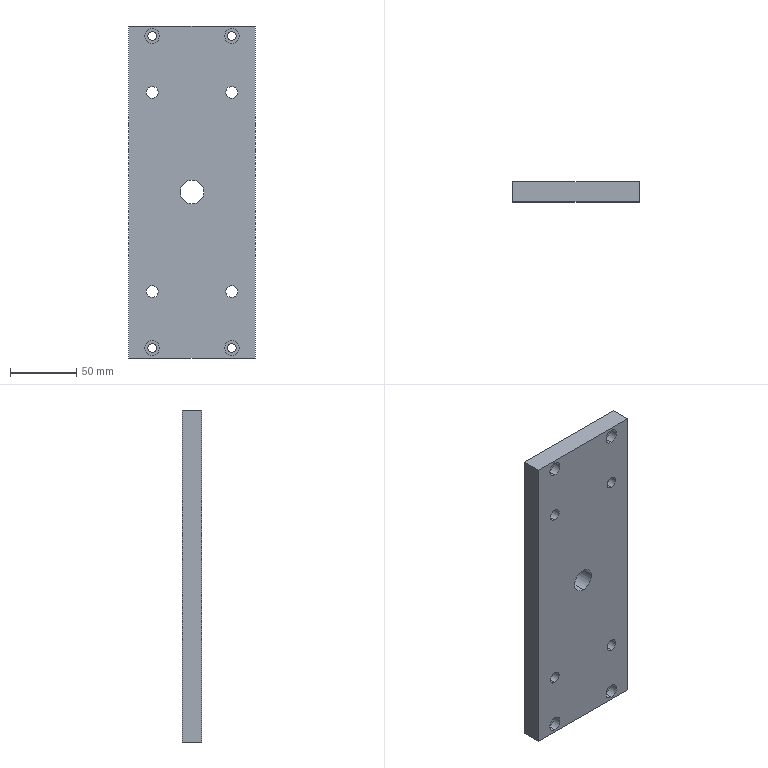Component | SolidWorks | 8TC-A15004-D0-01A-1 | 1 solid | 48 faces | box 95 x 15 x 250 mm | volume 341116 mm3 | cylinder 34 | plane 14 | commonest cylinder face diameters 15 x8 9 x8 11 x8 6.6 x8 18 x2 | material #45
build123d program:
from build123d import *

# Parameters (mm, degrees)
SKETCH1_W                                       = 95
SKETCH1_H                                       = 250
BOSS_EXTRUDE1_DEPTH                             = 7.5
M6_HEX_SOCKET_HEAD_CAP_SCREW_CBORE1_D           = 6.6
M6_HEX_SOCKET_HEAD_CAP_SCREW_CBORE1_DEPTH       = 15
M6_HEX_SOCKET_HEAD_CAP_SCREW_CBORE1_CBORE_D     = 11
M6_HEX_SOCKET_HEAD_CAP_SCREW_CBORE1_CBORE_DEPTH = 6.4
M6_HEX_SOCKET_HEAD_CAP_SCREW_CBORE1_TIP         = 1.983
M8_HEX_SOCKET_HEAD_CAP_SCREW_CBORE1_D           = 9
M8_HEX_SOCKET_HEAD_CAP_SCREW_CBORE1_CBORE_D     = 15
M8_HEX_SOCKET_HEAD_CAP_SCREW_CBORE1_CBORE_DEPTH = 8.6
SKETCH6_R                                       = 9
CUT_EXTRUDE1_DEPTH                              = 34


with BuildPart() as part:
    # Sketch1 → Boss-Extrude1 (new, symmetric)
    with BuildSketch(Plane(origin=(0, 0, 0), x_dir=(1, 0, 0), z_dir=(0, 1, 0))):
        Rectangle(SKETCH1_W, SKETCH1_H)
    extrude(amount=BOSS_EXTRUDE1_DEPTH, both=True)

    # M6 Hex Socket Head Cap Screw CBORE1
    with Locations(Plane(origin=(0, -7.5, 0), x_dir=(-1, 0, 0), z_dir=(0, -1, 0))):
        with Locations((-30, 117.5), (30, 117.5), (-30, -117.5), (30, -117.5)):
            CounterBoreHole(M6_HEX_SOCKET_HEAD_CAP_SCREW_CBORE1_D / 2, M6_HEX_SOCKET_HEAD_CAP_SCREW_CBORE1_CBORE_D / 2, M6_HEX_SOCKET_HEAD_CAP_SCREW_CBORE1_CBORE_DEPTH, depth=M6_HEX_SOCKET_HEAD_CAP_SCREW_CBORE1_DEPTH)
            with Locations((0, 0, -(M6_HEX_SOCKET_HEAD_CAP_SCREW_CBORE1_DEPTH + M6_HEX_SOCKET_HEAD_CAP_SCREW_CBORE1_TIP / 2))):  # 118° drill point
                Cone(0, M6_HEX_SOCKET_HEAD_CAP_SCREW_CBORE1_D / 2, M6_HEX_SOCKET_HEAD_CAP_SCREW_CBORE1_TIP, mode=Mode.SUBTRACT)

    # M8 Hex Socket Head Cap Screw CBORE1 (through all)
    with Locations(Plane(origin=(0, 7.5, 0), x_dir=(1, 0, 0), z_dir=(0, 1, 0))):
        with Locations((30, 75), (-30, 75), (-30, -75), (30, -75)):
            CounterBoreHole(M8_HEX_SOCKET_HEAD_CAP_SCREW_CBORE1_D / 2, M8_HEX_SOCKET_HEAD_CAP_SCREW_CBORE1_CBORE_D / 2, M8_HEX_SOCKET_HEAD_CAP_SCREW_CBORE1_CBORE_DEPTH)

    # Sketch6 → Cut-Extrude1 (cut)
    with BuildSketch(Plane(origin=(0, 7.5, 0), x_dir=(1, 0, 0), z_dir=(0, 1, 0))):
        with Locations(Location((0, 0, 0), (0, 0, 270))):
            Circle(SKETCH6_R)
    extrude(amount=-CUT_EXTRUDE1_DEPTH, mode=Mode.SUBTRACT)


solid = part.part